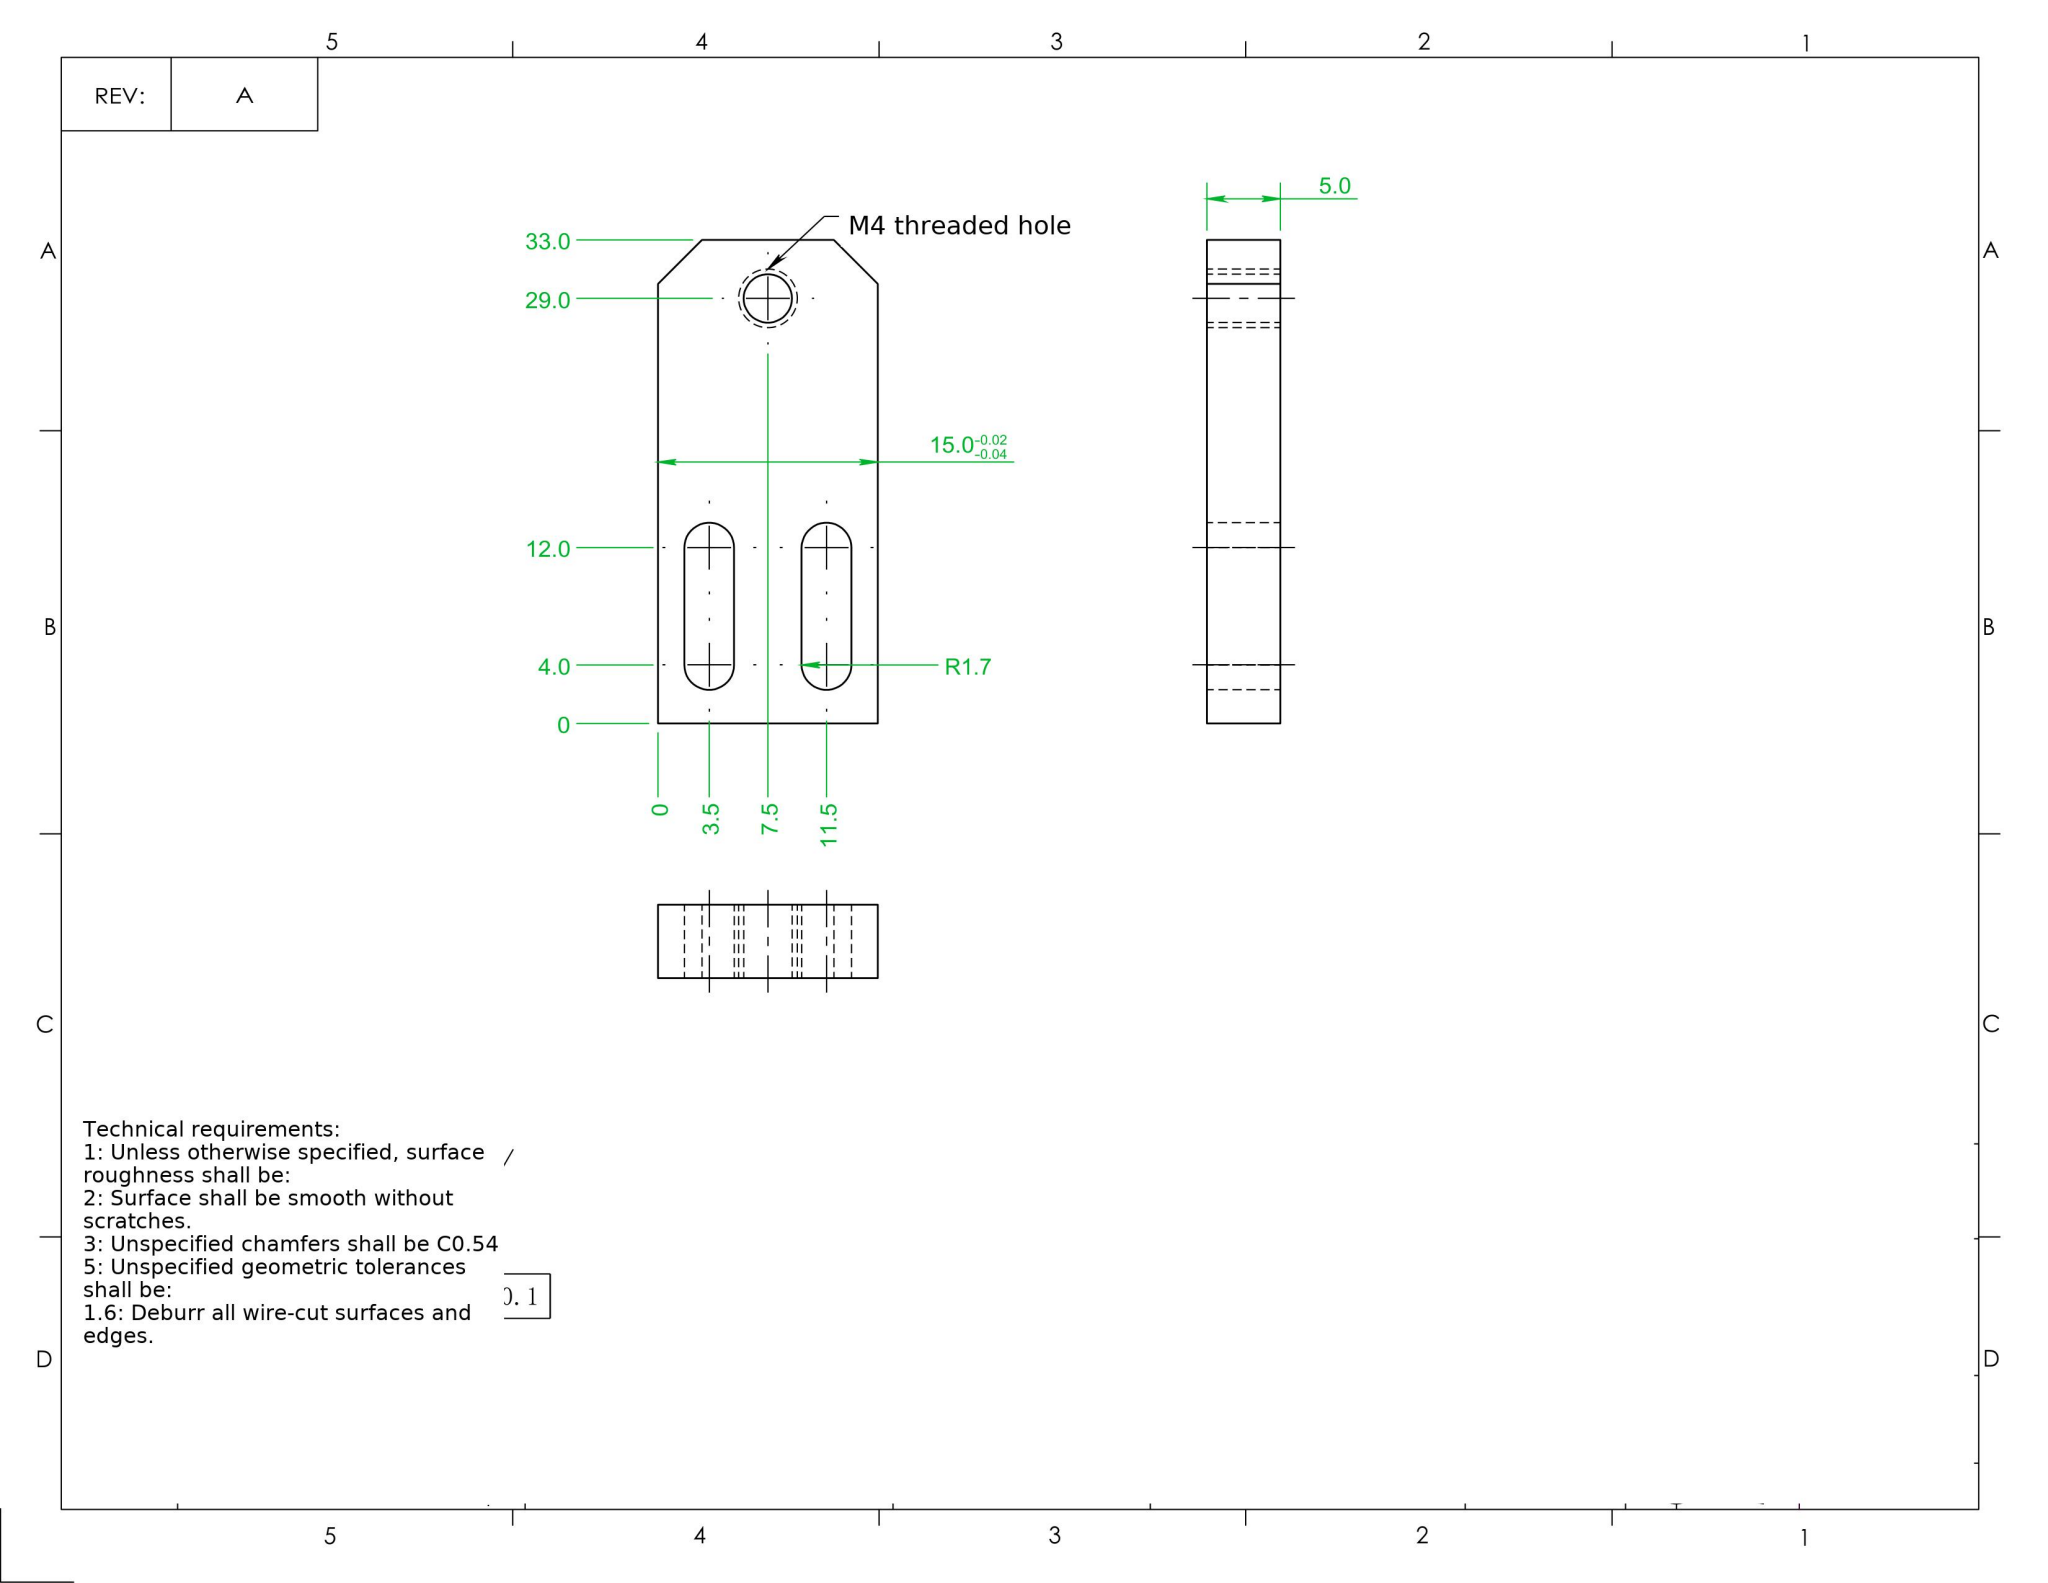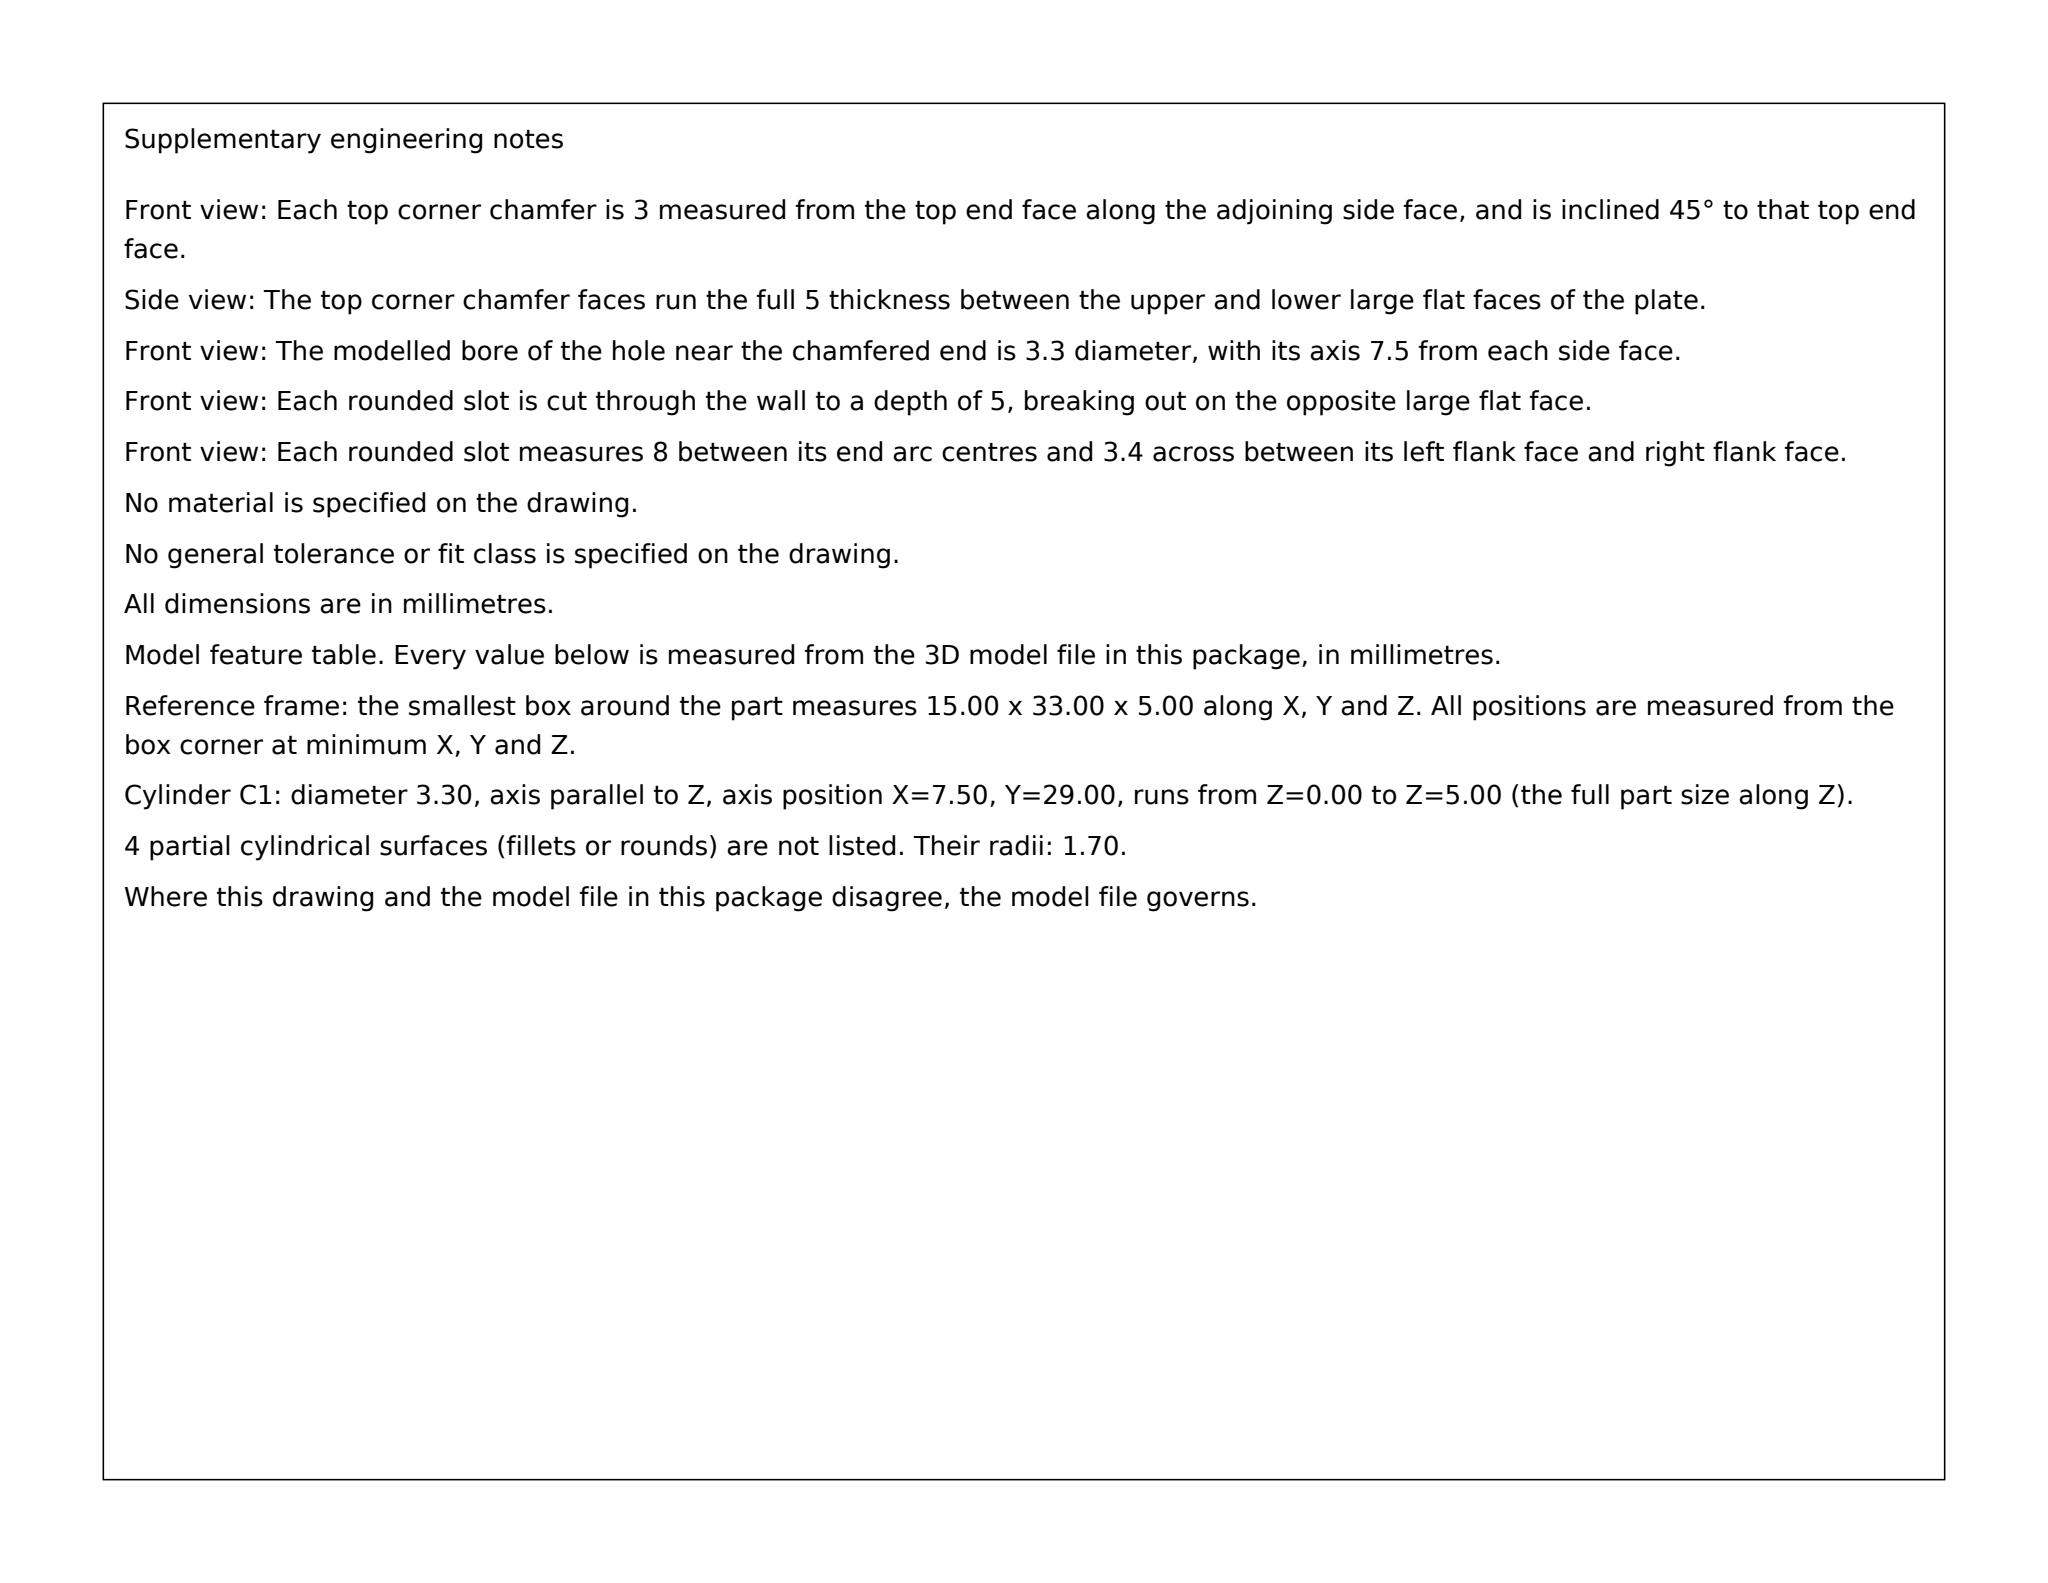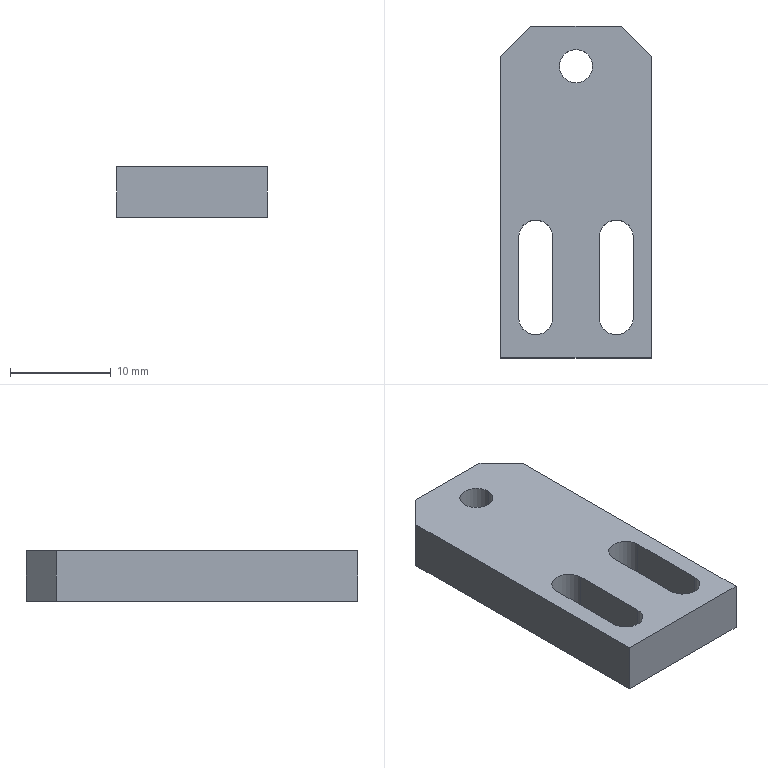Part | SolidWorks | mm | 1 solid | 18 faces | box 15 x 33 x 5 mm | volume 2024 mm3 | plane 12 | cylinder 6 | commonest cylinder face diameters 3.4 x4 3.3 x2
Drawing notes:
ALL DIMENSIONS IN MILLIMETERS (mm). | from the solid: STEP model facts stated in mm; bbox_xyz 15.0 x 33.0 x 5.0
M4 TAPPED HOLE THRU 5 THK (Ø3.3 TAP DRILL), LOCATED X7.5, Y29.0 FROM LOWER-LEFT CORNER OF PART | from the solid: cylinders[3.3,z,(7.5,29.0),length 5.0]
2X SLOT 3.4 WIDE, R1.7 ENDS, THRU 5 THK; SLOT AXES AT X3.5 AND X11.5, END CENTERS AT Y4.0 AND Y12.0 FROM LOWER-LEFT CORNER | from the solid: cylinders[3.4,z,(3.5,4.0),(3.5,12.0),(11.5,4.0),(11.5,12.0),length 5.0]; axis_planes x=1.8,5.2,9.8,13.2
PART OUTLINE 15.0 WIDE X 33.0 HIGH X 5.0 THICK, FACES AT X0/X15.0, Y0/Y33.0, Z0/Z5.0 | from the solid: bbox_xyz [15.0,33.0,5.0]; axis_planes x=0.0/15.0, y=0.0/33.0, z=0.0/5.0
build123d program:
from build123d import *

# Parameters (mm, degrees)
SKETCH1_W           = 15
SKETCH1_H           = 33
BOSS_EXTRUDE1_DEPTH = 13.4
SKETCH2_W           = 8.4
SKETCH2_H           = 33
CUT_EXTRUDE1_DEPTH  = 27.016
M4_TAPPED_HOLE1_D   = 3.3
CHAMFER1_SIZE       = 3
CUT_EXTRUDE2_DEPTH  = 19.802


with BuildPart() as part:
    # Sketch1 → Boss-Extrude1 (new body)
    with BuildSketch(Plane.XY):
        Rectangle(SKETCH1_W, SKETCH1_H)
    extrude(amount=BOSS_EXTRUDE1_DEPTH)

    # Sketch2 → Cut-Extrude1 (cut, through all)
    with BuildSketch(Plane.ZY.offset(7.5)):
        with Locations((9.2, 0)):
            Rectangle(SKETCH2_W, SKETCH2_H)
    extrude(amount=-CUT_EXTRUDE1_DEPTH, mode=Mode.SUBTRACT)

    # M4 Tapped Hole1 (through all)
    with Locations(Plane.XY.offset(5)):
        with Locations((0, 12.5)):
            Hole(M4_TAPPED_HOLE1_D / 2)

    # Chamfer1
    chamfer1_edges = [part.edges().sort_by_distance(p)[0] for p in [
        (-7.5, 16.5, 2.5),
        (7.5, 16.5, 2.5),
    ]]
    chamfer(chamfer1_edges, length=CHAMFER1_SIZE)

    # Sketch6 → Cut-Extrude2 (cut, through all)
    with BuildSketch(Plane(origin=(0, 0, 0), x_dir=(-1, 0, 0), z_dir=(0, 0, -1))):
        with BuildLine():
            Line((-2.3, -4.5), (-2.3, -12.5))
            ThreePointArc((-2.3, -12.5), (-4, -14.2), (-5.7, -12.5))
            Line((-5.7, -12.5), (-5.7, -4.5))
            ThreePointArc((-5.7, -4.5), (-4, -2.8), (-2.3, -4.5))
        make_face()
        with BuildLine():
            Line((2.3, -4.5), (2.3, -12.5))
            ThreePointArc((2.3, -12.5), (4, -14.2), (5.7, -12.5))
            Line((5.7, -12.5), (5.7, -4.5))
            ThreePointArc((5.7, -4.5), (4, -2.8), (2.3, -4.5))
        make_face()
    extrude(amount=-CUT_EXTRUDE2_DEPTH, mode=Mode.SUBTRACT)


solid = part.part
STEP:
#1=CARTESIAN_POINT('',(-1.65,12.5,0.));
#2=VERTEX_POINT('',#1);
#3=CARTESIAN_POINT('',(1.65,12.5,0.));
#4=VERTEX_POINT('',#3);
#5=CARTESIAN_POINT('',(0.,12.5,0.));
#6=DIRECTION('',(0.,0.,1.));
#7=DIRECTION('',(1.,0.,0.));
#8=AXIS2_PLACEMENT_3D('',#5,#6,#7);
#9=CIRCLE('',#8,1.65);
#10=EDGE_CURVE('',#2,#4,#9,.T.);
#11=ORIENTED_EDGE('',*,*,#10,.F.);
#12=CARTESIAN_POINT('',(-1.65,12.5,5.));
#13=VERTEX_POINT('',#12);
#14=CARTESIAN_POINT('',(-1.65,12.5,5.));
#15=DIRECTION('',(0.,0.,1.));
#16=VECTOR('',#15,1000.);
#17=LINE('',#14,#16);
#18=EDGE_CURVE('',#2,#13,#17,.T.);
#19=ORIENTED_EDGE('',*,*,#18,.T.);
#20=CARTESIAN_POINT('',(1.65,12.5,5.));
#21=VERTEX_POINT('',#20);
#22=CARTESIAN_POINT('',(0.,12.5,5.));
#23=DIRECTION('',(0.,0.,1.));
#24=DIRECTION('',(1.,0.,0.));
#25=AXIS2_PLACEMENT_3D('',#22,#23,#24);
#26=CIRCLE('',#25,1.65);
#27=EDGE_CURVE('',#13,#21,#26,.T.);
#28=ORIENTED_EDGE('',*,*,#27,.T.);
#29=CARTESIAN_POINT('',(1.65,12.5,5.));
#30=DIRECTION('',(0.,0.,1.));
#31=VECTOR('',#30,1000.);
#32=LINE('',#29,#31);
#33=EDGE_CURVE('',#4,#21,#32,.T.);
#34=ORIENTED_EDGE('',*,*,#33,.F.);
#35=EDGE_LOOP('',(#11,#19,#28,#34));
#36=FACE_OUTER_BOUND('',#35,.T.);
#37=CARTESIAN_POINT('',(0.,12.5,5.));
#38=DIRECTION('',(0.,0.,1.));
#39=DIRECTION('',(1.,0.,0.));
#40=AXIS2_PLACEMENT_3D('',#37,#38,#39);
#41=CYLINDRICAL_SURFACE('',#40,1.65);
#42=ADVANCED_FACE('',(#36),#41,.F.);
#43=CARTESIAN_POINT('',(7.5,-16.5,0.));
#44=VERTEX_POINT('',#43);
#45=CARTESIAN_POINT('',(7.5,13.5,0.));
#46=VERTEX_POINT('',#45);
#47=CARTESIAN_POINT('',(7.5,-16.5,0.));
#48=DIRECTION('',(0.,1.,0.));
#49=VECTOR('',#48,1000.);
#50=LINE('',#47,#49);
#51=EDGE_CURVE('',#44,#46,#50,.T.);
#52=ORIENTED_EDGE('',*,*,#51,.T.);
#53=CARTESIAN_POINT('',(7.5,13.5,5.));
#54=VERTEX_POINT('',#53);
#55=CARTESIAN_POINT('',(7.5,13.5,13.4));
#56=DIRECTION('',(0.,0.,1.));
#57=VECTOR('',#56,1000.);
#58=LINE('',#55,#57);
#59=EDGE_CURVE('',#46,#54,#58,.T.);
#60=ORIENTED_EDGE('',*,*,#59,.T.);
#61=CARTESIAN_POINT('',(7.5,-16.5,5.));
#62=VERTEX_POINT('',#61);
#63=CARTESIAN_POINT('',(7.5,16.5,5.));
#64=DIRECTION('',(0.,-1.,0.));
#65=VECTOR('',#64,1000.);
#66=LINE('',#63,#65);
#67=EDGE_CURVE('',#54,#62,#66,.T.);
#68=ORIENTED_EDGE('',*,*,#67,.T.);
#69=CARTESIAN_POINT('',(7.5,-16.5,13.4));
#70=DIRECTION('',(0.,0.,-1.));
#71=VECTOR('',#70,1000.);
#72=LINE('',#69,#71);
#73=EDGE_CURVE('',#62,#44,#72,.T.);
#74=ORIENTED_EDGE('',*,*,#73,.T.);
#75=EDGE_LOOP('',(#52,#60,#68,#74));
#76=FACE_OUTER_BOUND('',#75,.T.);
#77=CARTESIAN_POINT('',(7.5,-16.5,13.4));
#78=DIRECTION('',(-1.,0.,0.));
#79=DIRECTION('',(0.,0.,1.));
#80=AXIS2_PLACEMENT_3D('',#77,#78,#79);
#81=PLANE('',#80);
#82=ADVANCED_FACE('',(#76),#81,.F.);
#83=CARTESIAN_POINT('',(4.5,16.5,5.));
#84=VERTEX_POINT('',#83);
#85=CARTESIAN_POINT('',(-4.5,16.5,5.));
#86=VERTEX_POINT('',#85);
#87=CARTESIAN_POINT('',(7.5,16.5,5.));
#88=DIRECTION('',(-1.,0.,0.));
#89=VECTOR('',#88,1000.);
#90=LINE('',#87,#89);
#91=EDGE_CURVE('',#84,#86,#90,.T.);
#92=ORIENTED_EDGE('',*,*,#91,.F.);
#93=CARTESIAN_POINT('',(4.5,16.5,0.));
#94=VERTEX_POINT('',#93);
#95=CARTESIAN_POINT('',(4.5,16.5,13.4));
#96=DIRECTION('',(0.,0.,-1.));
#97=VECTOR('',#96,1000.);
#98=LINE('',#95,#97);
#99=EDGE_CURVE('',#84,#94,#98,.T.);
#100=ORIENTED_EDGE('',*,*,#99,.T.);
#101=CARTESIAN_POINT('',(-4.5,16.5,0.));
#102=VERTEX_POINT('',#101);
#103=CARTESIAN_POINT('',(-7.5,16.5,0.));
#104=DIRECTION('',(-1.,0.,0.));
#105=VECTOR('',#104,1000.);
#106=LINE('',#103,#105);
#107=EDGE_CURVE('',#94,#102,#106,.T.);
#108=ORIENTED_EDGE('',*,*,#107,.T.);
#109=CARTESIAN_POINT('',(-4.5,16.5,13.4));
#110=DIRECTION('',(0.,0.,1.));
#111=VECTOR('',#110,1000.);
#112=LINE('',#109,#111);
#113=EDGE_CURVE('',#102,#86,#112,.T.);
#114=ORIENTED_EDGE('',*,*,#113,.T.);
#115=EDGE_LOOP('',(#92,#100,#108,#114));
#116=FACE_OUTER_BOUND('',#115,.T.);
#117=CARTESIAN_POINT('',(-7.5,16.5,13.4));
#118=DIRECTION('',(0.,-1.,0.));
#119=DIRECTION('',(0.,0.,-1.));
#120=AXIS2_PLACEMENT_3D('',#117,#118,#119);
#121=PLANE('',#120);
#122=ADVANCED_FACE('',(#116),#121,.F.);
#123=CARTESIAN_POINT('',(-7.5,13.5,5.));
#124=VERTEX_POINT('',#123);
#125=CARTESIAN_POINT('',(-7.5,-16.5,5.));
#126=VERTEX_POINT('',#125);
#127=CARTESIAN_POINT('',(-7.5,16.5,5.));
#128=DIRECTION('',(0.,-1.,0.));
#129=VECTOR('',#128,1000.);
#130=LINE('',#127,#129);
#131=EDGE_CURVE('',#124,#126,#130,.T.);
#132=ORIENTED_EDGE('',*,*,#131,.F.);
#133=CARTESIAN_POINT('',(-7.5,13.5,0.));
#134=VERTEX_POINT('',#133);
#135=CARTESIAN_POINT('',(-7.5,13.5,13.4));
#136=DIRECTION('',(0.,0.,-1.));
#137=VECTOR('',#136,1000.);
#138=LINE('',#135,#137);
#139=EDGE_CURVE('',#124,#134,#138,.T.);
#140=ORIENTED_EDGE('',*,*,#139,.T.);
#141=CARTESIAN_POINT('',(-7.5,-16.5,0.));
#142=VERTEX_POINT('',#141);
#143=CARTESIAN_POINT('',(-7.5,-16.5,0.));
#144=DIRECTION('',(0.,-1.,0.));
#145=VECTOR('',#144,1000.);
#146=LINE('',#143,#145);
#147=EDGE_CURVE('',#134,#142,#146,.T.);
#148=ORIENTED_EDGE('',*,*,#147,.T.);
#149=CARTESIAN_POINT('',(-7.5,-16.5,13.4));
#150=DIRECTION('',(0.,0.,-1.));
#151=VECTOR('',#150,1000.);
#152=LINE('',#149,#151);
#153=EDGE_CURVE('',#126,#142,#152,.T.);
#154=ORIENTED_EDGE('',*,*,#153,.F.);
#155=EDGE_LOOP('',(#132,#140,#148,#154));
#156=FACE_OUTER_BOUND('',#155,.T.);
#157=CARTESIAN_POINT('',(-7.5,-16.5,13.4));
#158=DIRECTION('',(1.,0.,0.));
#159=DIRECTION('',(0.,0.,-1.));
#160=AXIS2_PLACEMENT_3D('',#157,#158,#159);
#161=PLANE('',#160);
#162=ADVANCED_FACE('',(#156),#161,.F.);
#163=ORIENTED_EDGE('',*,*,#73,.F.);
#164=CARTESIAN_POINT('',(7.5,-16.5,5.));
#165=DIRECTION('',(-1.,0.,0.));
#166=VECTOR('',#165,1000.);
#167=LINE('',#164,#166);
#168=EDGE_CURVE('',#62,#126,#167,.T.);
#169=ORIENTED_EDGE('',*,*,#168,.T.);
#170=ORIENTED_EDGE('',*,*,#153,.T.);
#171=CARTESIAN_POINT('',(-7.5,-16.5,0.));
#172=DIRECTION('',(1.,0.,0.));
#173=VECTOR('',#172,1000.);
#174=LINE('',#171,#173);
#175=EDGE_CURVE('',#142,#44,#174,.T.);
#176=ORIENTED_EDGE('',*,*,#175,.T.);
#177=EDGE_LOOP('',(#163,#169,#170,#176));
#178=FACE_OUTER_BOUND('',#177,.T.);
#179=CARTESIAN_POINT('',(-7.5,-16.5,13.4));
#180=DIRECTION('',(0.,1.,0.));
#181=DIRECTION('',(0.,0.,1.));
#182=AXIS2_PLACEMENT_3D('',#179,#180,#181);
#183=PLANE('',#182);
#184=ADVANCED_FACE('',(#178),#183,.F.);
#185=CARTESIAN_POINT('',(-5.7,-4.5,0.));
#186=VERTEX_POINT('',#185);
#187=CARTESIAN_POINT('',(-2.3,-4.5,0.));
#188=VERTEX_POINT('',#187);
#189=CARTESIAN_POINT('',(-4.,-4.5,0.));
#190=DIRECTION('',(0.,0.,-1.));
#191=DIRECTION('',(1.,0.,0.));
#192=AXIS2_PLACEMENT_3D('',#189,#190,#191);
#193=CIRCLE('',#192,1.7);
#194=EDGE_CURVE('',#186,#188,#193,.T.);
#195=ORIENTED_EDGE('',*,*,#194,.F.);
#196=CARTESIAN_POINT('',(-5.7,-12.5,0.));
#197=VERTEX_POINT('',#196);
#198=CARTESIAN_POINT('',(-5.7,-4.5,0.));
#199=DIRECTION('',(0.,1.,0.));
#200=VECTOR('',#199,1000.);
#201=LINE('',#198,#200);
#202=EDGE_CURVE('',#197,#186,#201,.T.);
#203=ORIENTED_EDGE('',*,*,#202,.F.);
#204=CARTESIAN_POINT('',(-2.3,-12.5,0.));
#205=VERTEX_POINT('',#204);
#206=CARTESIAN_POINT('',(-4.,-12.5,0.));
#207=DIRECTION('',(0.,0.,-1.));
#208=DIRECTION('',(1.,0.,0.));
#209=AXIS2_PLACEMENT_3D('',#206,#207,#208);
#210=CIRCLE('',#209,1.7);
#211=EDGE_CURVE('',#205,#197,#210,.T.);
#212=ORIENTED_EDGE('',*,*,#211,.F.);
#213=CARTESIAN_POINT('',(-2.3,-4.5,0.));
#214=DIRECTION('',(0.,-1.,0.));
#215=VECTOR('',#214,1000.);
#216=LINE('',#213,#215);
#217=EDGE_CURVE('',#188,#205,#216,.T.);
#218=ORIENTED_EDGE('',*,*,#217,.F.);
#219=EDGE_LOOP('',(#195,#203,#212,#218));
#220=FACE_BOUND('',#219,.T.);
#221=CARTESIAN_POINT('',(2.3,-4.5,0.));
#222=VERTEX_POINT('',#221);
#223=CARTESIAN_POINT('',(5.7,-4.5,0.));
#224=VERTEX_POINT('',#223);
#225=CARTESIAN_POINT('',(4.,-4.5,0.));
#226=DIRECTION('',(0.,0.,-1.));
#227=DIRECTION('',(-1.,0.,0.));
#228=AXIS2_PLACEMENT_3D('',#225,#226,#227);
#229=CIRCLE('',#228,1.7);
#230=EDGE_CURVE('',#222,#224,#229,.T.);
#231=ORIENTED_EDGE('',*,*,#230,.F.);
#232=CARTESIAN_POINT('',(2.3,-12.5,0.));
#233=VERTEX_POINT('',#232);
#234=CARTESIAN_POINT('',(2.3,-4.5,0.));
#235=DIRECTION('',(0.,1.,0.));
#236=VECTOR('',#235,1000.);
#237=LINE('',#234,#236);
#238=EDGE_CURVE('',#233,#222,#237,.T.);
#239=ORIENTED_EDGE('',*,*,#238,.F.);
#240=CARTESIAN_POINT('',(5.7,-12.5,0.));
#241=VERTEX_POINT('',#240);
#242=CARTESIAN_POINT('',(4.,-12.5,0.));
#243=DIRECTION('',(0.,0.,-1.));
#244=DIRECTION('',(-1.,0.,0.));
#245=AXIS2_PLACEMENT_3D('',#242,#243,#244);
#246=CIRCLE('',#245,1.7);
#247=EDGE_CURVE('',#241,#233,#246,.T.);
#248=ORIENTED_EDGE('',*,*,#247,.F.);
#249=CARTESIAN_POINT('',(5.7,-4.5,0.));
#250=DIRECTION('',(0.,-1.,0.));
#251=VECTOR('',#250,1000.);
#252=LINE('',#249,#251);
#253=EDGE_CURVE('',#224,#241,#252,.T.);
#254=ORIENTED_EDGE('',*,*,#253,.F.);
#255=EDGE_LOOP('',(#231,#239,#248,#254));
#256=FACE_BOUND('',#255,.T.);
#257=CARTESIAN_POINT('',(0.,12.5,0.));
#258=DIRECTION('',(0.,0.,1.));
#259=DIRECTION('',(1.,0.,0.));
#260=AXIS2_PLACEMENT_3D('',#257,#258,#259);
#261=CIRCLE('',#260,1.65);
#262=EDGE_CURVE('',#4,#2,#261,.T.);
#263=ORIENTED_EDGE('',*,*,#262,.T.);
#264=ORIENTED_EDGE('',*,*,#10,.T.);
#265=EDGE_LOOP('',(#263,#264));
#266=FACE_BOUND('',#265,.T.);
#267=ORIENTED_EDGE('',*,*,#107,.F.);
#268=CARTESIAN_POINT('',(10.5,10.5,0.));
#269=DIRECTION('',(0.7071,-0.7071,0.));
#270=VECTOR('',#269,1000.);
#271=LINE('',#268,#270);
#272=EDGE_CURVE('',#94,#46,#271,.T.);
#273=ORIENTED_EDGE('',*,*,#272,.T.);
#274=ORIENTED_EDGE('',*,*,#51,.F.);
#275=ORIENTED_EDGE('',*,*,#175,.F.);
#276=ORIENTED_EDGE('',*,*,#147,.F.);
#277=CARTESIAN_POINT('',(-10.5,10.5,0.));
#278=DIRECTION('',(0.7071,0.7071,0.));
#279=VECTOR('',#278,1000.);
#280=LINE('',#277,#279);
#281=EDGE_CURVE('',#134,#102,#280,.T.);
#282=ORIENTED_EDGE('',*,*,#281,.T.);
#283=EDGE_LOOP('',(#267,#273,#274,#275,#276,#282));
#284=FACE_OUTER_BOUND('',#283,.T.);
#285=CARTESIAN_POINT('',(0.,0.,0.));
#286=DIRECTION('',(0.,0.,-1.));
#287=DIRECTION('',(-1.,0.,0.));
#288=AXIS2_PLACEMENT_3D('',#285,#286,#287);
#289=PLANE('',#288);
#290=ADVANCED_FACE('',(#220,#256,#266,#284),#289,.T.);
#291=CARTESIAN_POINT('',(-5.7,-12.5,5.));
#292=VERTEX_POINT('',#291);
#293=CARTESIAN_POINT('',(-5.7,-4.5,5.));
#294=VERTEX_POINT('',#293);
#295=CARTESIAN_POINT('',(-5.7,-4.5,5.));
#296=DIRECTION('',(0.,1.,0.));
#297=VECTOR('',#296,1000.);
#298=LINE('',#295,#297);
#299=EDGE_CURVE('',#292,#294,#298,.T.);
#300=ORIENTED_EDGE('',*,*,#299,.T.);
#301=CARTESIAN_POINT('',(-2.3,-4.5,5.));
#302=VERTEX_POINT('',#301);
#303=CARTESIAN_POINT('',(-4.,-4.5,5.));
#304=DIRECTION('',(0.,0.,-1.));
#305=DIRECTION('',(1.,0.,0.));
#306=AXIS2_PLACEMENT_3D('',#303,#304,#305);
#307=CIRCLE('',#306,1.7);
#308=EDGE_CURVE('',#294,#302,#307,.T.);
#309=ORIENTED_EDGE('',*,*,#308,.T.);
#310=CARTESIAN_POINT('',(-2.3,-12.5,5.));
#311=VERTEX_POINT('',#310);
#312=CARTESIAN_POINT('',(-2.3,-4.5,5.));
#313=DIRECTION('',(0.,-1.,0.));
#314=VECTOR('',#313,1000.);
#315=LINE('',#312,#314);
#316=EDGE_CURVE('',#302,#311,#315,.T.);
#317=ORIENTED_EDGE('',*,*,#316,.T.);
#318=CARTESIAN_POINT('',(-4.,-12.5,5.));
#319=DIRECTION('',(0.,0.,-1.));
#320=DIRECTION('',(1.,0.,0.));
#321=AXIS2_PLACEMENT_3D('',#318,#319,#320);
#322=CIRCLE('',#321,1.7);
#323=EDGE_CURVE('',#311,#292,#322,.T.);
#324=ORIENTED_EDGE('',*,*,#323,.T.);
#325=EDGE_LOOP('',(#300,#309,#317,#324));
#326=FACE_BOUND('',#325,.T.);
#327=CARTESIAN_POINT('',(2.3,-12.5,5.));
#328=VERTEX_POINT('',#327);
#329=CARTESIAN_POINT('',(2.3,-4.5,5.));
#330=VERTEX_POINT('',#329);
#331=CARTESIAN_POINT('',(2.3,-4.5,5.));
#332=DIRECTION('',(0.,1.,0.));
#333=VECTOR('',#332,1000.);
#334=LINE('',#331,#333);
#335=EDGE_CURVE('',#328,#330,#334,.T.);
#336=ORIENTED_EDGE('',*,*,#335,.T.);
#337=CARTESIAN_POINT('',(5.7,-4.5,5.));
#338=VERTEX_POINT('',#337);
#339=CARTESIAN_POINT('',(4.,-4.5,5.));
#340=DIRECTION('',(0.,0.,-1.));
#341=DIRECTION('',(-1.,0.,0.));
#342=AXIS2_PLACEMENT_3D('',#339,#340,#341);
#343=CIRCLE('',#342,1.7);
#344=EDGE_CURVE('',#330,#338,#343,.T.);
#345=ORIENTED_EDGE('',*,*,#344,.T.);
#346=CARTESIAN_POINT('',(5.7,-12.5,5.));
#347=VERTEX_POINT('',#346);
#348=CARTESIAN_POINT('',(5.7,-4.5,5.));
#349=DIRECTION('',(0.,-1.,0.));
#350=VECTOR('',#349,1000.);
#351=LINE('',#348,#350);
#352=EDGE_CURVE('',#338,#347,#351,.T.);
#353=ORIENTED_EDGE('',*,*,#352,.T.);
#354=CARTESIAN_POINT('',(4.,-12.5,5.));
#355=DIRECTION('',(0.,0.,-1.));
#356=DIRECTION('',(-1.,0.,0.));
#357=AXIS2_PLACEMENT_3D('',#354,#355,#356);
#358=CIRCLE('',#357,1.7);
#359=EDGE_CURVE('',#347,#328,#358,.T.);
#360=ORIENTED_EDGE('',*,*,#359,.T.);
#361=EDGE_LOOP('',(#336,#345,#353,#360));
#362=FACE_BOUND('',#361,.T.);
#363=CARTESIAN_POINT('',(0.,12.5,5.));
#364=DIRECTION('',(0.,0.,1.));
#365=DIRECTION('',(1.,0.,0.));
#366=AXIS2_PLACEMENT_3D('',#363,#364,#365);
#367=CIRCLE('',#366,1.65);
#368=EDGE_CURVE('',#21,#13,#367,.T.);
#369=ORIENTED_EDGE('',*,*,#368,.F.);
#370=ORIENTED_EDGE('',*,*,#27,.F.);
#371=EDGE_LOOP('',(#369,#370));
#372=FACE_BOUND('',#371,.T.);
#373=ORIENTED_EDGE('',*,*,#67,.F.);
#374=CARTESIAN_POINT('',(4.5,16.5,5.));
#375=DIRECTION('',(-0.7071,0.7071,-0.));
#376=VECTOR('',#375,1000.);
#377=LINE('',#374,#376);
#378=EDGE_CURVE('',#54,#84,#377,.T.);
#379=ORIENTED_EDGE('',*,*,#378,.T.);
#380=ORIENTED_EDGE('',*,*,#91,.T.);
#381=CARTESIAN_POINT('',(-7.5,13.5,5.));
#382=DIRECTION('',(-0.7071,-0.7071,0.));
#383=VECTOR('',#382,1000.);
#384=LINE('',#381,#383);
#385=EDGE_CURVE('',#86,#124,#384,.T.);
#386=ORIENTED_EDGE('',*,*,#385,.T.);
#387=ORIENTED_EDGE('',*,*,#131,.T.);
#388=ORIENTED_EDGE('',*,*,#168,.F.);
#389=EDGE_LOOP('',(#373,#379,#380,#386,#387,#388));
#390=FACE_OUTER_BOUND('',#389,.T.);
#391=CARTESIAN_POINT('',(7.5,16.5,5.));
#392=DIRECTION('',(0.,-0.,-1.));
#393=DIRECTION('',(0.,1.,-0.));
#394=AXIS2_PLACEMENT_3D('',#391,#392,#393);
#395=PLANE('',#394);
#396=ADVANCED_FACE('',(#326,#362,#372,#390),#395,.F.);
#397=ORIENTED_EDGE('',*,*,#18,.F.);
#398=ORIENTED_EDGE('',*,*,#262,.F.);
#399=ORIENTED_EDGE('',*,*,#33,.T.);
#400=ORIENTED_EDGE('',*,*,#368,.T.);
#401=EDGE_LOOP('',(#397,#398,#399,#400));
#402=FACE_OUTER_BOUND('',#401,.T.);
#403=CARTESIAN_POINT('',(0.,12.5,5.));
#404=DIRECTION('',(0.,0.,1.));
#405=DIRECTION('',(1.,0.,0.));
#406=AXIS2_PLACEMENT_3D('',#403,#404,#405);
#407=CYLINDRICAL_SURFACE('',#406,1.65);
#408=ADVANCED_FACE('',(#402),#407,.F.);
#409=ORIENTED_EDGE('',*,*,#378,.F.);
#410=ORIENTED_EDGE('',*,*,#59,.F.);
#411=ORIENTED_EDGE('',*,*,#272,.F.);
#412=ORIENTED_EDGE('',*,*,#99,.F.);
#413=EDGE_LOOP('',(#409,#410,#411,#412));
#414=FACE_OUTER_BOUND('',#413,.T.);
#415=CARTESIAN_POINT('',(4.5,16.5,13.4));
#416=DIRECTION('',(-0.7071,-0.7071,0.));
#417=DIRECTION('',(0.,0.,-1.));
#418=AXIS2_PLACEMENT_3D('',#415,#416,#417);
#419=PLANE('',#418);
#420=ADVANCED_FACE('',(#414),#419,.F.);
#421=ORIENTED_EDGE('',*,*,#385,.F.);
#422=ORIENTED_EDGE('',*,*,#113,.F.);
#423=ORIENTED_EDGE('',*,*,#281,.F.);
#424=ORIENTED_EDGE('',*,*,#139,.F.);
#425=EDGE_LOOP('',(#421,#422,#423,#424));
#426=FACE_OUTER_BOUND('',#425,.T.);
#427=CARTESIAN_POINT('',(-7.5,13.5,13.4));
#428=DIRECTION('',(0.7071,-0.7071,0.));
#429=DIRECTION('',(0.,0.,-1.));
#430=AXIS2_PLACEMENT_3D('',#427,#428,#429);
#431=PLANE('',#430);
#432=ADVANCED_FACE('',(#426),#431,.F.);
#433=ORIENTED_EDGE('',*,*,#230,.T.);
#434=CARTESIAN_POINT('',(5.7,-4.5,5.));
#435=DIRECTION('',(0.,0.,-1.));
#436=VECTOR('',#435,1000.);
#437=LINE('',#434,#436);
#438=EDGE_CURVE('',#338,#224,#437,.T.);
#439=ORIENTED_EDGE('',*,*,#438,.F.);
#440=ORIENTED_EDGE('',*,*,#344,.F.);
#441=CARTESIAN_POINT('',(2.3,-4.5,5.));
#442=DIRECTION('',(0.,0.,-1.));
#443=VECTOR('',#442,1000.);
#444=LINE('',#441,#443);
#445=EDGE_CURVE('',#330,#222,#444,.T.);
#446=ORIENTED_EDGE('',*,*,#445,.T.);
#447=EDGE_LOOP('',(#433,#439,#440,#446));
#448=FACE_OUTER_BOUND('',#447,.T.);
#449=CARTESIAN_POINT('',(4.,-4.5,5.));
#450=DIRECTION('',(0.,0.,-1.));
#451=DIRECTION('',(-1.,0.,0.));
#452=AXIS2_PLACEMENT_3D('',#449,#450,#451);
#453=CYLINDRICAL_SURFACE('',#452,1.7);
#454=ADVANCED_FACE('',(#448),#453,.F.);
#455=ORIENTED_EDGE('',*,*,#238,.T.);
#456=ORIENTED_EDGE('',*,*,#445,.F.);
#457=ORIENTED_EDGE('',*,*,#335,.F.);
#458=CARTESIAN_POINT('',(2.3,-12.5,5.));
#459=DIRECTION('',(0.,0.,-1.));
#460=VECTOR('',#459,1000.);
#461=LINE('',#458,#460);
#462=EDGE_CURVE('',#328,#233,#461,.T.);
#463=ORIENTED_EDGE('',*,*,#462,.T.);
#464=EDGE_LOOP('',(#455,#456,#457,#463));
#465=FACE_OUTER_BOUND('',#464,.T.);
#466=CARTESIAN_POINT('',(2.3,-4.5,5.));
#467=DIRECTION('',(-1.,0.,0.));
#468=DIRECTION('',(0.,0.,1.));
#469=AXIS2_PLACEMENT_3D('',#466,#467,#468);
#470=PLANE('',#469);
#471=ADVANCED_FACE('',(#465),#470,.F.);
#472=ORIENTED_EDGE('',*,*,#247,.T.);
#473=ORIENTED_EDGE('',*,*,#462,.F.);
#474=ORIENTED_EDGE('',*,*,#359,.F.);
#475=CARTESIAN_POINT('',(5.7,-12.5,5.));
#476=DIRECTION('',(0.,0.,-1.));
#477=VECTOR('',#476,1000.);
#478=LINE('',#475,#477);
#479=EDGE_CURVE('',#347,#241,#478,.T.);
#480=ORIENTED_EDGE('',*,*,#479,.T.);
#481=EDGE_LOOP('',(#472,#473,#474,#480));
#482=FACE_OUTER_BOUND('',#481,.T.);
#483=CARTESIAN_POINT('',(4.,-12.5,5.));
#484=DIRECTION('',(0.,0.,-1.));
#485=DIRECTION('',(-1.,0.,0.));
#486=AXIS2_PLACEMENT_3D('',#483,#484,#485);
#487=CYLINDRICAL_SURFACE('',#486,1.7);
#488=ADVANCED_FACE('',(#482),#487,.F.);
#489=ORIENTED_EDGE('',*,*,#253,.T.);
#490=ORIENTED_EDGE('',*,*,#479,.F.);
#491=ORIENTED_EDGE('',*,*,#352,.F.);
#492=ORIENTED_EDGE('',*,*,#438,.T.);
#493=EDGE_LOOP('',(#489,#490,#491,#492));
#494=FACE_OUTER_BOUND('',#493,.T.);
#495=CARTESIAN_POINT('',(5.7,-4.5,5.));
#496=DIRECTION('',(1.,0.,0.));
#497=DIRECTION('',(0.,0.,-1.));
#498=AXIS2_PLACEMENT_3D('',#495,#496,#497);
#499=PLANE('',#498);
#500=ADVANCED_FACE('',(#494),#499,.F.);
#501=ORIENTED_EDGE('',*,*,#194,.T.);
#502=CARTESIAN_POINT('',(-2.3,-4.5,5.));
#503=DIRECTION('',(0.,0.,-1.));
#504=VECTOR('',#503,1000.);
#505=LINE('',#502,#504);
#506=EDGE_CURVE('',#302,#188,#505,.T.);
#507=ORIENTED_EDGE('',*,*,#506,.F.);
#508=ORIENTED_EDGE('',*,*,#308,.F.);
#509=CARTESIAN_POINT('',(-5.7,-4.5,5.));
#510=DIRECTION('',(0.,0.,-1.));
#511=VECTOR('',#510,1000.);
#512=LINE('',#509,#511);
#513=EDGE_CURVE('',#294,#186,#512,.T.);
#514=ORIENTED_EDGE('',*,*,#513,.T.);
#515=EDGE_LOOP('',(#501,#507,#508,#514));
#516=FACE_OUTER_BOUND('',#515,.T.);
#517=CARTESIAN_POINT('',(-4.,-4.5,5.));
#518=DIRECTION('',(0.,0.,-1.));
#519=DIRECTION('',(-1.,0.,0.));
#520=AXIS2_PLACEMENT_3D('',#517,#518,#519);
#521=CYLINDRICAL_SURFACE('',#520,1.7);
#522=ADVANCED_FACE('',(#516),#521,.F.);
#523=ORIENTED_EDGE('',*,*,#202,.T.);
#524=ORIENTED_EDGE('',*,*,#513,.F.);
#525=ORIENTED_EDGE('',*,*,#299,.F.);
#526=CARTESIAN_POINT('',(-5.7,-12.5,5.));
#527=DIRECTION('',(0.,0.,-1.));
#528=VECTOR('',#527,1000.);
#529=LINE('',#526,#528);
#530=EDGE_CURVE('',#292,#197,#529,.T.);
#531=ORIENTED_EDGE('',*,*,#530,.T.);
#532=EDGE_LOOP('',(#523,#524,#525,#531));
#533=FACE_OUTER_BOUND('',#532,.T.);
#534=CARTESIAN_POINT('',(-5.7,-4.5,5.));
#535=DIRECTION('',(-1.,0.,0.));
#536=DIRECTION('',(-0.,-1.,0.));
#537=AXIS2_PLACEMENT_3D('',#534,#535,#536);
#538=PLANE('',#537);
#539=ADVANCED_FACE('',(#533),#538,.F.);
#540=ORIENTED_EDGE('',*,*,#211,.T.);
#541=ORIENTED_EDGE('',*,*,#530,.F.);
#542=ORIENTED_EDGE('',*,*,#323,.F.);
#543=CARTESIAN_POINT('',(-2.3,-12.5,5.));
#544=DIRECTION('',(0.,0.,-1.));
#545=VECTOR('',#544,1000.);
#546=LINE('',#543,#545);
#547=EDGE_CURVE('',#311,#205,#546,.T.);
#548=ORIENTED_EDGE('',*,*,#547,.T.);
#549=EDGE_LOOP('',(#540,#541,#542,#548));
#550=FACE_OUTER_BOUND('',#549,.T.);
#551=CARTESIAN_POINT('',(-4.,-12.5,5.));
#552=DIRECTION('',(0.,0.,-1.));
#553=DIRECTION('',(-1.,0.,0.));
#554=AXIS2_PLACEMENT_3D('',#551,#552,#553);
#555=CYLINDRICAL_SURFACE('',#554,1.7);
#556=ADVANCED_FACE('',(#550),#555,.F.);
#557=ORIENTED_EDGE('',*,*,#217,.T.);
#558=ORIENTED_EDGE('',*,*,#547,.F.);
#559=ORIENTED_EDGE('',*,*,#316,.F.);
#560=ORIENTED_EDGE('',*,*,#506,.T.);
#561=EDGE_LOOP('',(#557,#558,#559,#560));
#562=FACE_OUTER_BOUND('',#561,.T.);
#563=CARTESIAN_POINT('',(-2.3,-4.5,5.));
#564=DIRECTION('',(1.,0.,0.));
#565=DIRECTION('',(0.,0.,-1.));
#566=AXIS2_PLACEMENT_3D('',#563,#564,#565);
#567=PLANE('',#566);
#568=ADVANCED_FACE('',(#562),#567,.F.);
#569=CLOSED_SHELL('',(#42,#82,#122,#162,#184,#290,#396,#408,#420,#432,#454,#471,#488,#500,#522,#539,#556,#568));
#570=MANIFOLD_SOLID_BREP('',#569);
#571=CARTESIAN_POINT('',(0.,0.,0.));
#572=DIRECTION('',(0.,0.,1.));
#573=DIRECTION('',(1.,0.,0.));
#574=AXIS2_PLACEMENT_3D('',#571,#572,#573);
#575=(LENGTH_UNIT()NAMED_UNIT(*)SI_UNIT(.MILLI.,.METRE.));
#576=UNCERTAINTY_MEASURE_WITH_UNIT(LENGTH_MEASURE(0.00001),#575,'','');
#577=(NAMED_UNIT(*)PLANE_ANGLE_UNIT()SI_UNIT($,.RADIAN.));
#578=(NAMED_UNIT(*)SI_UNIT($,.STERADIAN.)SOLID_ANGLE_UNIT());
#579=(GEOMETRIC_REPRESENTATION_CONTEXT(3)GLOBAL_UNCERTAINTY_ASSIGNED_CONTEXT((#576))GLOBAL_UNIT_ASSIGNED_CONTEXT((#575,#577,#578))REPRESENTATION_CONTEXT('',''));
#580=ADVANCED_BREP_SHAPE_REPRESENTATION('',(#570,#574),#579);